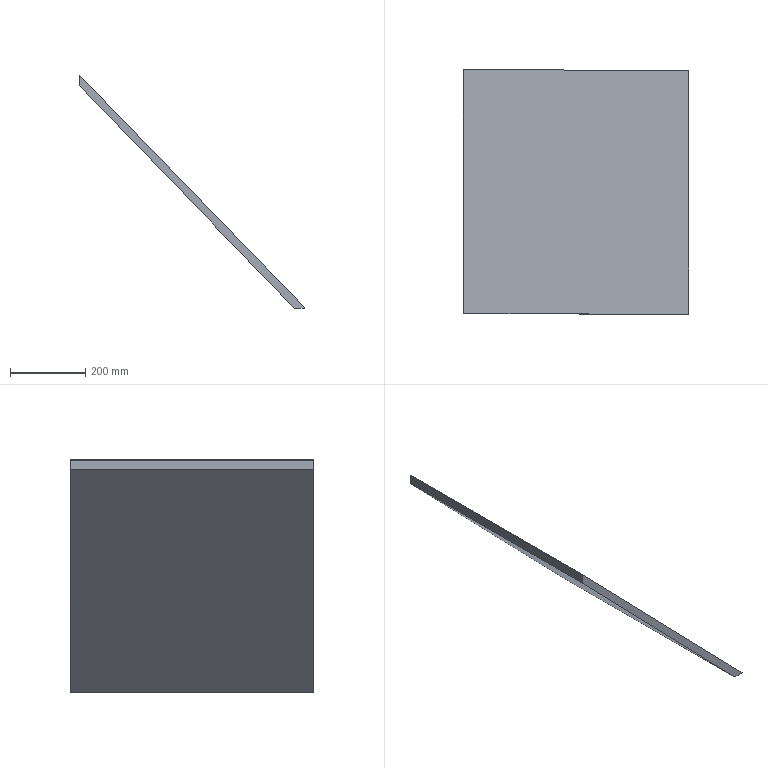Component | SolidWorks | ElectromagneticBeamBasePlate3-1 | 1 solid | 8 faces | box 601 x 650 x 620.93 mm | volume 10992050 mm3 | plane 8 | material Plain Carbon Steel
STEP:
#1=COLOUR_RGB('',0.7922,0.8196,0.9333);
#2=FILL_AREA_STYLE_COLOUR('',#1);
#3=FILL_AREA_STYLE('',(#2));
#4=SURFACE_STYLE_FILL_AREA(#3);
#5=SURFACE_SIDE_STYLE('',(#4));
#6=SURFACE_STYLE_USAGE(.BOTH.,#5);
#7=PRESENTATION_STYLE_ASSIGNMENT((#6));
#8=CARTESIAN_POINT('',(-236.081,140.226,239.842));
#9=VERTEX_POINT('',#8);
#10=CARTESIAN_POINT('',(-236.081,140.226,238.831));
#11=VERTEX_POINT('',#10);
#12=CARTESIAN_POINT('',(-236.081,140.226,214.966));
#13=DIRECTION('',(-0.,0.,-1.));
#14=VECTOR('',#13,39.37);
#15=LINE('',#12,#14);
#16=EDGE_CURVE('',#9,#11,#15,.T.);
#17=ORIENTED_EDGE('',*,*,#16,.F.);
#18=CARTESIAN_POINT('',(-236.02,140.226,239.901));
#19=VERTEX_POINT('',#18);
#20=CARTESIAN_POINT('',(-236.586,140.226,239.353));
#21=DIRECTION('',(0.7186,-0.,0.6954));
#22=VECTOR('',#21,39.37);
#23=LINE('',#20,#22);
#24=EDGE_CURVE('',#9,#19,#23,.T.);
#25=ORIENTED_EDGE('',*,*,#24,.T.);
#26=CARTESIAN_POINT('',(-212.42,140.226,215.514));
#27=VERTEX_POINT('',#26);
#28=CARTESIAN_POINT('',(-212.42,140.226,215.514));
#29=DIRECTION('',(-0.6954,-0.,0.7186));
#30=VECTOR('',#29,39.37);
#31=LINE('',#28,#30);
#32=EDGE_CURVE('',#27,#19,#31,.T.);
#33=ORIENTED_EDGE('',*,*,#32,.F.);
#34=CARTESIAN_POINT('',(-212.481,140.226,215.455));
#35=VERTEX_POINT('',#34);
#36=CARTESIAN_POINT('',(-212.986,140.226,214.966));
#37=DIRECTION('',(0.7186,-0.,0.6954));
#38=VECTOR('',#37,39.37);
#39=LINE('',#36,#38);
#40=EDGE_CURVE('',#35,#27,#39,.T.);
#41=ORIENTED_EDGE('',*,*,#40,.F.);
#42=CARTESIAN_POINT('',(-213.491,140.226,215.488));
#43=VERTEX_POINT('',#42);
#44=CARTESIAN_POINT('',(-212.969,140.226,215.471));
#45=DIRECTION('',(0.9995,0.,-0.03278));
#46=VECTOR('',#45,39.37);
#47=LINE('',#44,#46);
#48=EDGE_CURVE('',#43,#35,#47,.T.);
#49=ORIENTED_EDGE('',*,*,#48,.F.);
#50=CARTESIAN_POINT('',(-212.986,140.226,214.966));
#51=DIRECTION('',(-0.6954,-0.,0.7186));
#52=VECTOR('',#51,39.37);
#53=LINE('',#50,#52);
#54=EDGE_CURVE('',#43,#11,#53,.T.);
#55=ORIENTED_EDGE('',*,*,#54,.T.);
#56=EDGE_LOOP('',(#17,#25,#33,#41,#49,#55));
#57=FACE_OUTER_BOUND('',#56,.T.);
#58=CARTESIAN_POINT('',(-212.986,140.226,214.966));
#59=DIRECTION('',(-0.,1.,0.));
#60=DIRECTION('',(-0.6954,-0.,0.7186));
#61=AXIS2_PLACEMENT_3D('',#58,#59,#60);
#62=PLANE('',#61);
#63=ADVANCED_FACE('',(#57),#62,.T.);
#64=CARTESIAN_POINT('',(-212.481,114.635,215.455));
#65=VERTEX_POINT('',#64);
#66=CARTESIAN_POINT('',(-212.481,140.226,215.455));
#67=DIRECTION('',(0.,-1.,-0.));
#68=VECTOR('',#67,39.37);
#69=LINE('',#66,#68);
#70=EDGE_CURVE('',#35,#65,#69,.T.);
#71=ORIENTED_EDGE('',*,*,#70,.F.);
#72=ORIENTED_EDGE('',*,*,#40,.T.);
#73=CARTESIAN_POINT('',(-212.42,114.635,215.514));
#74=VERTEX_POINT('',#73);
#75=CARTESIAN_POINT('',(-212.42,140.226,215.514));
#76=DIRECTION('',(-0.,1.,0.));
#77=VECTOR('',#76,39.37);
#78=LINE('',#75,#77);
#79=EDGE_CURVE('',#74,#27,#78,.T.);
#80=ORIENTED_EDGE('',*,*,#79,.F.);
#81=CARTESIAN_POINT('',(-212.986,114.635,214.966));
#82=DIRECTION('',(0.7186,-0.,0.6954));
#83=VECTOR('',#82,39.37);
#84=LINE('',#81,#83);
#85=EDGE_CURVE('',#65,#74,#84,.T.);
#86=ORIENTED_EDGE('',*,*,#85,.F.);
#87=EDGE_LOOP('',(#71,#72,#80,#86));
#88=FACE_OUTER_BOUND('',#87,.T.);
#89=CARTESIAN_POINT('',(-212.986,140.226,214.966));
#90=DIRECTION('',(0.6954,0.,-0.7186));
#91=DIRECTION('',(-0.,1.,0.));
#92=AXIS2_PLACEMENT_3D('',#89,#90,#91);
#93=PLANE('',#92);
#94=ADVANCED_FACE('',(#88),#93,.T.);
#95=CARTESIAN_POINT('',(-236.081,114.635,238.831));
#96=VERTEX_POINT('',#95);
#97=CARTESIAN_POINT('',(-236.081,114.635,239.842));
#98=VERTEX_POINT('',#97);
#99=CARTESIAN_POINT('',(-236.081,114.635,214.966));
#100=DIRECTION('',(0.,-0.,1.));
#101=VECTOR('',#100,39.37);
#102=LINE('',#99,#101);
#103=EDGE_CURVE('',#96,#98,#102,.T.);
#104=ORIENTED_EDGE('',*,*,#103,.F.);
#105=CARTESIAN_POINT('',(-213.491,114.635,215.488));
#106=VERTEX_POINT('',#105);
#107=CARTESIAN_POINT('',(-212.986,114.635,214.966));
#108=DIRECTION('',(0.6954,0.,-0.7186));
#109=VECTOR('',#108,39.37);
#110=LINE('',#107,#109);
#111=EDGE_CURVE('',#96,#106,#110,.T.);
#112=ORIENTED_EDGE('',*,*,#111,.T.);
#113=CARTESIAN_POINT('',(-212.969,114.635,215.471));
#114=DIRECTION('',(-0.9995,-0.,0.03278));
#115=VECTOR('',#114,39.37);
#116=LINE('',#113,#115);
#117=EDGE_CURVE('',#65,#106,#116,.T.);
#118=ORIENTED_EDGE('',*,*,#117,.F.);
#119=ORIENTED_EDGE('',*,*,#85,.T.);
#120=CARTESIAN_POINT('',(-236.02,114.635,239.901));
#121=VERTEX_POINT('',#120);
#122=CARTESIAN_POINT('',(-212.42,114.635,215.514));
#123=DIRECTION('',(0.6954,0.,-0.7186));
#124=VECTOR('',#123,39.37);
#125=LINE('',#122,#124);
#126=EDGE_CURVE('',#121,#74,#125,.T.);
#127=ORIENTED_EDGE('',*,*,#126,.F.);
#128=CARTESIAN_POINT('',(-236.586,114.635,239.353));
#129=DIRECTION('',(0.7186,-0.,0.6954));
#130=VECTOR('',#129,39.37);
#131=LINE('',#128,#130);
#132=EDGE_CURVE('',#98,#121,#131,.T.);
#133=ORIENTED_EDGE('',*,*,#132,.F.);
#134=EDGE_LOOP('',(#104,#112,#118,#119,#127,#133));
#135=FACE_OUTER_BOUND('',#134,.T.);
#136=CARTESIAN_POINT('',(-212.986,114.635,214.966));
#137=DIRECTION('',(0.,-1.,-0.));
#138=DIRECTION('',(0.6954,0.,-0.7186));
#139=AXIS2_PLACEMENT_3D('',#136,#137,#138);
#140=PLANE('',#139);
#141=ADVANCED_FACE('',(#135),#140,.T.);
#142=CARTESIAN_POINT('',(-236.081,140.226,239.842));
#143=DIRECTION('',(-0.,1.,0.));
#144=VECTOR('',#143,39.37);
#145=LINE('',#142,#144);
#146=EDGE_CURVE('',#98,#9,#145,.T.);
#147=ORIENTED_EDGE('',*,*,#146,.F.);
#148=ORIENTED_EDGE('',*,*,#132,.T.);
#149=CARTESIAN_POINT('',(-236.02,140.226,239.901));
#150=DIRECTION('',(0.,-1.,-0.));
#151=VECTOR('',#150,39.37);
#152=LINE('',#149,#151);
#153=EDGE_CURVE('',#19,#121,#152,.T.);
#154=ORIENTED_EDGE('',*,*,#153,.F.);
#155=ORIENTED_EDGE('',*,*,#24,.F.);
#156=EDGE_LOOP('',(#147,#148,#154,#155));
#157=FACE_OUTER_BOUND('',#156,.T.);
#158=CARTESIAN_POINT('',(-236.586,140.226,239.353));
#159=DIRECTION('',(-0.6954,-0.,0.7186));
#160=DIRECTION('',(0.,-1.,-0.));
#161=AXIS2_PLACEMENT_3D('',#158,#159,#160);
#162=PLANE('',#161);
#163=ADVANCED_FACE('',(#157),#162,.T.);
#164=ORIENTED_EDGE('',*,*,#111,.F.);
#165=CARTESIAN_POINT('',(-236.081,140.226,238.831));
#166=DIRECTION('',(-0.,1.,0.));
#167=VECTOR('',#166,39.37);
#168=LINE('',#165,#167);
#169=EDGE_CURVE('',#96,#11,#168,.T.);
#170=ORIENTED_EDGE('',*,*,#169,.T.);
#171=ORIENTED_EDGE('',*,*,#54,.F.);
#172=CARTESIAN_POINT('',(-213.491,140.226,215.488));
#173=DIRECTION('',(0.,-1.,-0.));
#174=VECTOR('',#173,39.37);
#175=LINE('',#172,#174);
#176=EDGE_CURVE('',#43,#106,#175,.T.);
#177=ORIENTED_EDGE('',*,*,#176,.T.);
#178=EDGE_LOOP('',(#164,#170,#171,#177));
#179=FACE_OUTER_BOUND('',#178,.T.);
#180=CARTESIAN_POINT('',(-212.986,140.226,214.966));
#181=DIRECTION('',(0.7186,-0.,0.6954));
#182=DIRECTION('',(-0.6954,-0.,0.7186));
#183=AXIS2_PLACEMENT_3D('',#180,#181,#182);
#184=PLANE('',#183);
#185=ADVANCED_FACE('',(#179),#184,.F.);
#186=ORIENTED_EDGE('',*,*,#32,.T.);
#187=ORIENTED_EDGE('',*,*,#153,.T.);
#188=ORIENTED_EDGE('',*,*,#126,.T.);
#189=ORIENTED_EDGE('',*,*,#79,.T.);
#190=EDGE_LOOP('',(#186,#187,#188,#189));
#191=FACE_OUTER_BOUND('',#190,.T.);
#192=CARTESIAN_POINT('',(-212.42,140.226,215.514));
#193=DIRECTION('',(0.7186,-0.,0.6954));
#194=DIRECTION('',(-0.6954,-0.,0.7186));
#195=AXIS2_PLACEMENT_3D('',#192,#193,#194);
#196=PLANE('',#195);
#197=ADVANCED_FACE('',(#191),#196,.T.);
#198=ORIENTED_EDGE('',*,*,#48,.T.);
#199=ORIENTED_EDGE('',*,*,#70,.T.);
#200=ORIENTED_EDGE('',*,*,#117,.T.);
#201=ORIENTED_EDGE('',*,*,#176,.F.);
#202=EDGE_LOOP('',(#198,#199,#200,#201));
#203=FACE_OUTER_BOUND('',#202,.T.);
#204=CARTESIAN_POINT('',(-212.076,169.753,215.441));
#205=DIRECTION('',(0.03278,-0.,0.9995));
#206=DIRECTION('',(-0.9995,-0.,0.03278));
#207=AXIS2_PLACEMENT_3D('',#204,#205,#206);
#208=PLANE('',#207);
#209=ADVANCED_FACE('',(#203),#208,.F.);
#210=ORIENTED_EDGE('',*,*,#146,.T.);
#211=ORIENTED_EDGE('',*,*,#16,.T.);
#212=ORIENTED_EDGE('',*,*,#169,.F.);
#213=ORIENTED_EDGE('',*,*,#103,.T.);
#214=EDGE_LOOP('',(#210,#211,#212,#213));
#215=FACE_OUTER_BOUND('',#214,.T.);
#216=CARTESIAN_POINT('',(-236.081,169.753,240.247));
#217=DIRECTION('',(1.,0.,-0.));
#218=DIRECTION('',(0.,-0.,1.));
#219=AXIS2_PLACEMENT_3D('',#216,#217,#218);
#220=PLANE('',#219);
#221=ADVANCED_FACE('',(#215),#220,.F.);
#222=CLOSED_SHELL('',(#63,#94,#141,#163,#185,#197,#209,#221));
#223=MANIFOLD_SOLID_BREP('',#222);
#224=STYLED_ITEM('',(#7),#223);
#225=PRESENTATION_LAYER_ASSIGNMENT('','',(#224));
#226=(LENGTH_UNIT()NAMED_UNIT(*)SI_UNIT($,.METRE.));
#227=LENGTH_MEASURE_WITH_UNIT(LENGTH_MEASURE(0.0254),#226);
#228=DIMENSIONAL_EXPONENTS(1.,0.,0.,0.,0.,0.,0.);
#229=(CONVERSION_BASED_UNIT('',#227)LENGTH_UNIT()NAMED_UNIT(#228));
#230=UNCERTAINTY_MEASURE_WITH_UNIT(LENGTH_MEASURE(0.00001),#229,'','');
#231=(NAMED_UNIT(*)PLANE_ANGLE_UNIT()SI_UNIT($,.RADIAN.));
#232=(NAMED_UNIT(*)SI_UNIT($,.STERADIAN.)SOLID_ANGLE_UNIT());
#233=(GEOMETRIC_REPRESENTATION_CONTEXT(3)GLOBAL_UNCERTAINTY_ASSIGNED_CONTEXT((#230))GLOBAL_UNIT_ASSIGNED_CONTEXT((#229,#231,#232))REPRESENTATION_CONTEXT('',''));
#234=MECHANICAL_DESIGN_GEOMETRIC_PRESENTATION_REPRESENTATION('',(#224),#233);
#235=CARTESIAN_POINT('',(0.,0.,0.));
#236=DIRECTION('',(0.,0.,1.));
#237=DIRECTION('',(1.,0.,0.));
#238=AXIS2_PLACEMENT_3D('',#235,#236,#237);
#239=(LENGTH_UNIT()NAMED_UNIT(*)SI_UNIT($,.METRE.));
#240=LENGTH_MEASURE_WITH_UNIT(LENGTH_MEASURE(0.0254),#239);
#241=DIMENSIONAL_EXPONENTS(1.,0.,0.,0.,0.,0.,0.);
#242=(CONVERSION_BASED_UNIT('',#240)LENGTH_UNIT()NAMED_UNIT(#241));
#243=UNCERTAINTY_MEASURE_WITH_UNIT(LENGTH_MEASURE(0.00001),#242,'','');
#244=(NAMED_UNIT(*)PLANE_ANGLE_UNIT()SI_UNIT($,.RADIAN.));
#245=(NAMED_UNIT(*)SI_UNIT($,.STERADIAN.)SOLID_ANGLE_UNIT());
#246=(GEOMETRIC_REPRESENTATION_CONTEXT(3)GLOBAL_UNCERTAINTY_ASSIGNED_CONTEXT((#243))GLOBAL_UNIT_ASSIGNED_CONTEXT((#242,#244,#245))REPRESENTATION_CONTEXT('',''));
#247=ADVANCED_BREP_SHAPE_REPRESENTATION('',(#223,#238),#246);